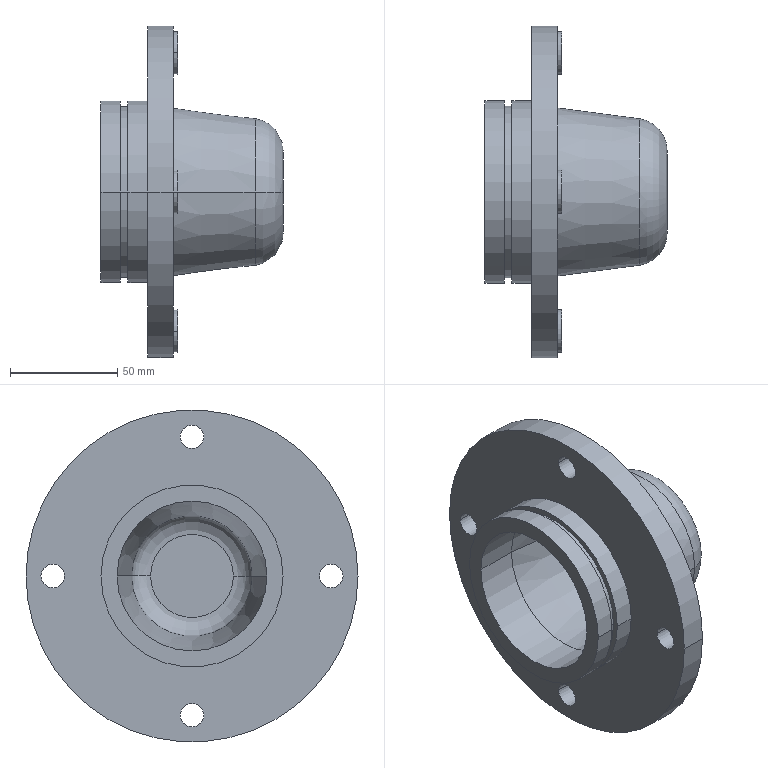Component | SolidWorks | 12RearCover-1 | 1 solid | 45 faces | box 85 x 155 x 155 mm | volume 290547 mm3 | cylinder 26 | plane 11 | cone 4 | torus 4 | commonest cylinder face diameters 11 x8 20 x8 85 x4 70 x2 80 x2 155 x2
build123d program:
from build123d import *

# Parameters (mm, degrees)
CUT_EXTRUDE2_START  = -12.575
SKETCH28_R          = 42.5
SKETCH28_R_2        = 40
CUT_EXTRUDE2_DEPTH  = 3.55
SKETCH29_R          = 10
BOSS_EXTRUDE3_DEPTH = 2
SKETCH30_R          = 5.5
CUT_EXTRUDE3_DEPTH  = 121.138
CIRPATTERN2_COUNT   = 4


with BuildPart() as part:
    # Sketch27 → Revolve2 (revolve)
    with BuildSketch(Plane(origin=(0, 0, 0), x_dir=(0, 0, -1), z_dir=(1, 0, 0)), mode=Mode.PRIVATE) as revolve2_sk:
        with BuildLine():
            Line((0, 42.5), (-21.8, 42.5))
            Line((-21.8, 42.5), (-21.8, 77.5))
            Line((-21.8, 77.5), (-33.8, 77.5))
            Line((-33.8, 77.5), (-33.8, 39.25))
            Line((-33.8, 39.25), (-71.961, 34.219))
            ThreePointArc((-71.961, 34.219), (-81.278, 29.237), (-85, 19.348))
            Line((-85, 19.348), (-85, 0))
            Line((-85, 0), (-79, 0))
            Line((-79, 0), (-79, 19.348))
            ThreePointArc((-79, 19.348), (-76.767, 25.281), (-71.176, 28.271))
            Line((-71.176, 28.271), (-20.132, 35))
            Line((-20.132, 35), (0, 35))
            Line((0, 35), (0, 42.5))
        make_face()
    revolve(revolve2_sk.sketch.rotate(Axis((0, 0, 0), (0, 0, 1)), 90), axis=Axis((0, 0, 0), (0, 0, 1)))

    # Sketch28 → Cut-Extrude2 (cut)
    with BuildSketch(Plane(origin=(0, 0, 0), x_dir=(-1, 0, 0), z_dir=(0, 0, -1)).offset(CUT_EXTRUDE2_START)):
        Circle(SKETCH28_R)
        Circle(SKETCH28_R_2, mode=Mode.SUBTRACT)
    extrude(amount=CUT_EXTRUDE2_DEPTH, mode=Mode.SUBTRACT)

    # Sketch29 → Boss-Extrude3 (add)
    with BuildSketch(Plane.XY.offset(33.8)):
        with Locations((0, 65)):
            Circle(SKETCH29_R)
    boss_extrude3 = extrude(amount=BOSS_EXTRUDE3_DEPTH)

    # Sketch30 → Cut-Extrude3 (cut, through all)
    with BuildSketch(Plane.XY.offset(35.8)):
        with Locations((0, 65)):
            Circle(SKETCH30_R)
    cut_extrude3 = extrude(amount=-CUT_EXTRUDE3_DEPTH, mode=Mode.SUBTRACT)

    # CirPattern2: Boss-Extrude3, Cut-Extrude3 ×4 about axis
    cirpattern2_axis = Axis((0, 0, 0), (0, 0, 1))
    add([boss_extrude3.rotate(cirpattern2_axis, i * 360 / CIRPATTERN2_COUNT) for i in range(1, CIRPATTERN2_COUNT)])
    add([cut_extrude3.rotate(cirpattern2_axis, i * 360 / CIRPATTERN2_COUNT) for i in range(1, CIRPATTERN2_COUNT)], mode=Mode.SUBTRACT)


solid = part.part

# Placed as in the assembly
solid = solid.moved(Location((213.085, -90.191, 512), (0, 90, 0)))